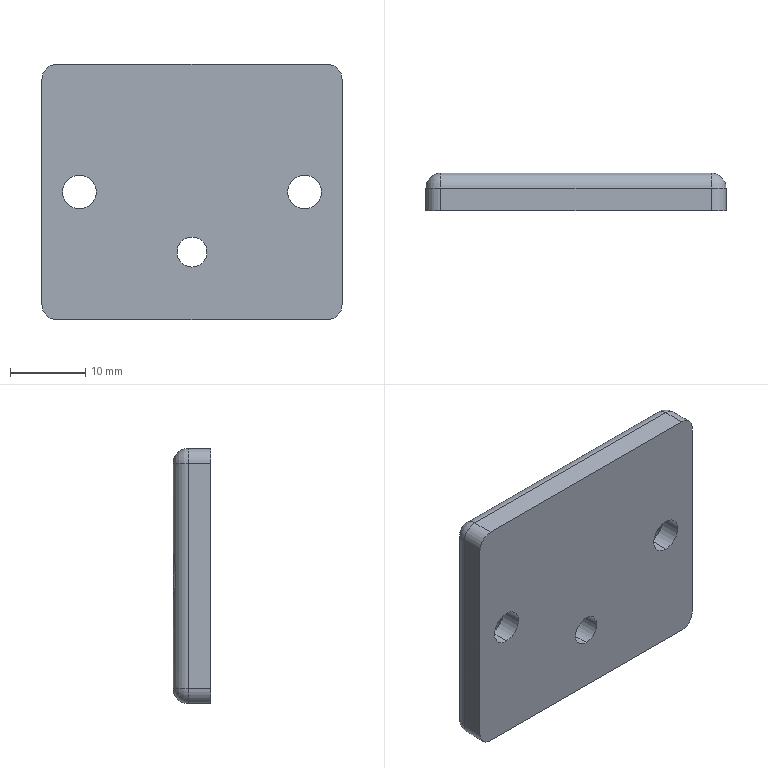Component | SolidWorks | 18ZTJ-NVT-01-006-1 | 1 solid | 28 faces | box 40 x 5 x 34 mm | volume 6347 mm3 | cylinder 14 | plane 6 | cone 4 | sphere 4 | commonest cylinder face diameters 4 x10 4.5 x4 | material #45
STEP:
#1=COLOUR_RGB('',0.7922,0.8196,0.9333);
#2=FILL_AREA_STYLE_COLOUR('',#1);
#3=FILL_AREA_STYLE('',(#2));
#4=SURFACE_STYLE_FILL_AREA(#3);
#5=SURFACE_SIDE_STYLE('',(#4));
#6=SURFACE_STYLE_USAGE(.BOTH.,#5);
#7=PRESENTATION_STYLE_ASSIGNMENT((#6));
#8=CARTESIAN_POINT('',(-0.5354,0.3728,3.583));
#9=VERTEX_POINT('',#8);
#10=CARTESIAN_POINT('',(-0.5354,0.3728,3.74));
#11=VERTEX_POINT('',#10);
#12=CARTESIAN_POINT('',(-0.5354,0.3728,3.661));
#13=DIRECTION('',(0.,1.,0.));
#14=DIRECTION('',(0.,0.,1.));
#15=AXIS2_PLACEMENT_3D('',#12,#13,#14);
#16=CIRCLE('',#15,0.07874);
#17=EDGE_CURVE('',#9,#11,#16,.T.);
#18=ORIENTED_EDGE('',*,*,#17,.F.);
#19=CARTESIAN_POINT('',(-0.5354,0.5697,3.583));
#20=VERTEX_POINT('',#19);
#21=CARTESIAN_POINT('',(-0.5354,0.5697,3.583));
#22=DIRECTION('',(0.,1.,0.));
#23=VECTOR('',#22,39.37);
#24=LINE('',#21,#23);
#25=EDGE_CURVE('',#9,#20,#24,.T.);
#26=ORIENTED_EDGE('',*,*,#25,.T.);
#27=CARTESIAN_POINT('',(-0.5354,0.5697,3.74));
#28=VERTEX_POINT('',#27);
#29=CARTESIAN_POINT('',(-0.5354,0.5697,3.661));
#30=DIRECTION('',(0.,1.,0.));
#31=DIRECTION('',(0.,0.,1.));
#32=AXIS2_PLACEMENT_3D('',#29,#30,#31);
#33=CIRCLE('',#32,0.07874);
#34=EDGE_CURVE('',#20,#28,#33,.T.);
#35=ORIENTED_EDGE('',*,*,#34,.T.);
#36=CARTESIAN_POINT('',(-0.5354,0.5697,3.74));
#37=DIRECTION('',(0.,1.,0.));
#38=VECTOR('',#37,39.37);
#39=LINE('',#36,#38);
#40=EDGE_CURVE('',#11,#28,#39,.T.);
#41=ORIENTED_EDGE('',*,*,#40,.F.);
#42=EDGE_LOOP('',(#18,#26,#35,#41));
#43=FACE_OUTER_BOUND('',#42,.T.);
#44=CARTESIAN_POINT('',(-0.5354,0.5697,3.661));
#45=DIRECTION('',(0.,1.,0.));
#46=DIRECTION('',(0.,0.,1.));
#47=AXIS2_PLACEMENT_3D('',#44,#45,#46);
#48=CYLINDRICAL_SURFACE('',#47,0.07874);
#49=ADVANCED_FACE('',(#43),#48,.F.);
#50=CARTESIAN_POINT('',(-1.126,0.4819,3.888));
#51=VERTEX_POINT('',#50);
#52=CARTESIAN_POINT('',(-1.126,0.4819,4.065));
#53=VERTEX_POINT('',#52);
#54=CARTESIAN_POINT('',(-1.126,0.4819,3.976));
#55=DIRECTION('',(0.,1.,0.));
#56=DIRECTION('',(0.,0.,1.));
#57=AXIS2_PLACEMENT_3D('',#54,#55,#56);
#58=CIRCLE('',#57,0.08858);
#59=EDGE_CURVE('',#51,#53,#58,.T.);
#60=ORIENTED_EDGE('',*,*,#59,.F.);
#61=CARTESIAN_POINT('',(-1.126,0.5697,3.8));
#62=VERTEX_POINT('',#61);
#63=CARTESIAN_POINT('',(-1.126,0.5697,3.8));
#64=DIRECTION('',(0.,0.7071,-0.7071));
#65=VECTOR('',#64,39.37);
#66=LINE('',#63,#65);
#67=EDGE_CURVE('',#51,#62,#66,.T.);
#68=ORIENTED_EDGE('',*,*,#67,.T.);
#69=CARTESIAN_POINT('',(-1.244,0.5697,3.845));
#70=VERTEX_POINT('',#69);
#71=CARTESIAN_POINT('',(-1.126,0.5697,3.976));
#72=DIRECTION('',(0.,1.,0.));
#73=DIRECTION('',(0.,0.,1.));
#74=AXIS2_PLACEMENT_3D('',#71,#72,#73);
#75=CIRCLE('',#74,0.1764);
#76=EDGE_CURVE('',#62,#70,#75,.T.);
#77=ORIENTED_EDGE('',*,*,#76,.T.);
#78=CARTESIAN_POINT('',(-1.244,0.5697,4.107));
#79=VERTEX_POINT('',#78);
#80=CARTESIAN_POINT('',(-1.244,0.5697,3.845));
#81=CARTESIAN_POINT('',(-1.249,0.5697,3.849));
#82=CARTESIAN_POINT('',(-1.253,0.5693,3.854));
#83=CARTESIAN_POINT('',(-1.26,0.5682,3.863));
#84=CARTESIAN_POINT('',(-1.263,0.5675,3.868));
#85=CARTESIAN_POINT('',(-1.268,0.5659,3.879));
#86=CARTESIAN_POINT('',(-1.271,0.565,3.884));
#87=CARTESIAN_POINT('',(-1.275,0.5633,3.895));
#88=CARTESIAN_POINT('',(-1.277,0.5624,3.901));
#89=CARTESIAN_POINT('',(-1.282,0.5599,3.917));
#90=CARTESIAN_POINT('',(-1.285,0.5585,3.929));
#91=CARTESIAN_POINT('',(-1.288,0.5565,3.953));
#92=CARTESIAN_POINT('',(-1.289,0.5559,3.964));
#93=CARTESIAN_POINT('',(-1.289,0.5559,3.988));
#94=CARTESIAN_POINT('',(-1.288,0.5565,4.));
#95=CARTESIAN_POINT('',(-1.285,0.5585,4.024));
#96=CARTESIAN_POINT('',(-1.282,0.5599,4.035));
#97=CARTESIAN_POINT('',(-1.277,0.5624,4.052));
#98=CARTESIAN_POINT('',(-1.275,0.5632,4.057));
#99=CARTESIAN_POINT('',(-1.271,0.565,4.068));
#100=CARTESIAN_POINT('',(-1.268,0.5659,4.074));
#101=CARTESIAN_POINT('',(-1.263,0.5675,4.084));
#102=CARTESIAN_POINT('',(-1.26,0.5682,4.089));
#103=CARTESIAN_POINT('',(-1.253,0.5693,4.099));
#104=CARTESIAN_POINT('',(-1.249,0.5697,4.103));
#105=CARTESIAN_POINT('',(-1.244,0.5697,4.107));
#106=B_SPLINE_CURVE_WITH_KNOTS('',3,(#80,#81,#82,#83,#84,#85,#86,#87,#88,#89,#90,#91,#92,#93,#94,#95,#96,#97,#98,#99,#100,#101,#102,#103,#104,#105),.UNSPECIFIED.,.F.,.F.,(4,2,2,2,2,2,2,2,2,2,2,2,4),(0.,0.000451,0.000902,0.001353,0.001804,0.002706,0.003608,0.00451,0.005412,0.005863,0.006314,0.006765,0.007216),.UNSPECIFIED.);
#107=EDGE_CURVE('',#70,#79,#106,.T.);
#108=ORIENTED_EDGE('',*,*,#107,.T.);
#109=CARTESIAN_POINT('',(-1.126,0.5697,4.153));
#110=VERTEX_POINT('',#109);
#111=CARTESIAN_POINT('',(-1.126,0.5697,3.976));
#112=DIRECTION('',(0.,1.,0.));
#113=DIRECTION('',(0.,0.,1.));
#114=AXIS2_PLACEMENT_3D('',#111,#112,#113);
#115=CIRCLE('',#114,0.1764);
#116=EDGE_CURVE('',#79,#110,#115,.T.);
#117=ORIENTED_EDGE('',*,*,#116,.T.);
#118=CARTESIAN_POINT('',(-1.126,0.5697,4.153));
#119=DIRECTION('',(0.,0.7071,0.7071));
#120=VECTOR('',#119,39.37);
#121=LINE('',#118,#120);
#122=EDGE_CURVE('',#53,#110,#121,.T.);
#123=ORIENTED_EDGE('',*,*,#122,.F.);
#124=EDGE_LOOP('',(#60,#68,#77,#108,#117,#123));
#125=FACE_OUTER_BOUND('',#124,.T.);
#126=CARTESIAN_POINT('',(-1.126,0.5697,3.976));
#127=DIRECTION('',(0.,1.,0.));
#128=DIRECTION('',(0.,0.,1.));
#129=AXIS2_PLACEMENT_3D('',#126,#127,#128);
#130=CONICAL_SURFACE('',#129,0.1764,0.7854);
#131=ADVANCED_FACE('',(#125),#130,.F.);
#132=CARTESIAN_POINT('',(-1.126,0.3728,3.888));
#133=VERTEX_POINT('',#132);
#134=CARTESIAN_POINT('',(-1.126,0.3728,4.065));
#135=VERTEX_POINT('',#134);
#136=CARTESIAN_POINT('',(-1.126,0.3728,3.976));
#137=DIRECTION('',(0.,1.,0.));
#138=DIRECTION('',(0.,0.,1.));
#139=AXIS2_PLACEMENT_3D('',#136,#137,#138);
#140=CIRCLE('',#139,0.08858);
#141=EDGE_CURVE('',#133,#135,#140,.T.);
#142=ORIENTED_EDGE('',*,*,#141,.F.);
#143=CARTESIAN_POINT('',(-1.126,0.5697,3.888));
#144=DIRECTION('',(0.,1.,0.));
#145=VECTOR('',#144,39.37);
#146=LINE('',#143,#145);
#147=EDGE_CURVE('',#133,#51,#146,.T.);
#148=ORIENTED_EDGE('',*,*,#147,.T.);
#149=ORIENTED_EDGE('',*,*,#59,.T.);
#150=CARTESIAN_POINT('',(-1.126,0.5697,4.065));
#151=DIRECTION('',(0.,1.,0.));
#152=VECTOR('',#151,39.37);
#153=LINE('',#150,#152);
#154=EDGE_CURVE('',#135,#53,#153,.T.);
#155=ORIENTED_EDGE('',*,*,#154,.F.);
#156=EDGE_LOOP('',(#142,#148,#149,#155));
#157=FACE_OUTER_BOUND('',#156,.T.);
#158=CARTESIAN_POINT('',(-1.126,0.5697,3.976));
#159=DIRECTION('',(0.,1.,0.));
#160=DIRECTION('',(0.,0.,1.));
#161=AXIS2_PLACEMENT_3D('',#158,#159,#160);
#162=CYLINDRICAL_SURFACE('',#161,0.08858);
#163=ADVANCED_FACE('',(#157),#162,.F.);
#164=CARTESIAN_POINT('',(0.05513,0.4819,3.888));
#165=VERTEX_POINT('',#164);
#166=CARTESIAN_POINT('',(0.05513,0.4819,4.065));
#167=VERTEX_POINT('',#166);
#168=CARTESIAN_POINT('',(0.05513,0.4819,3.976));
#169=DIRECTION('',(0.,1.,0.));
#170=DIRECTION('',(0.,0.,1.));
#171=AXIS2_PLACEMENT_3D('',#168,#169,#170);
#172=CIRCLE('',#171,0.08858);
#173=EDGE_CURVE('',#165,#167,#172,.T.);
#174=ORIENTED_EDGE('',*,*,#173,.F.);
#175=CARTESIAN_POINT('',(0.05513,0.5697,3.8));
#176=VERTEX_POINT('',#175);
#177=CARTESIAN_POINT('',(0.05513,0.5697,3.8));
#178=DIRECTION('',(0.,0.7071,-0.7071));
#179=VECTOR('',#178,39.37);
#180=LINE('',#177,#179);
#181=EDGE_CURVE('',#165,#176,#180,.T.);
#182=ORIENTED_EDGE('',*,*,#181,.T.);
#183=CARTESIAN_POINT('',(0.05513,0.5697,4.153));
#184=VERTEX_POINT('',#183);
#185=CARTESIAN_POINT('',(0.05513,0.5697,3.976));
#186=DIRECTION('',(0.,1.,0.));
#187=DIRECTION('',(0.,0.,1.));
#188=AXIS2_PLACEMENT_3D('',#185,#186,#187);
#189=CIRCLE('',#188,0.1764);
#190=EDGE_CURVE('',#176,#184,#189,.T.);
#191=ORIENTED_EDGE('',*,*,#190,.T.);
#192=CARTESIAN_POINT('',(0.05513,0.5697,4.153));
#193=DIRECTION('',(0.,0.7071,0.7071));
#194=VECTOR('',#193,39.37);
#195=LINE('',#192,#194);
#196=EDGE_CURVE('',#167,#184,#195,.T.);
#197=ORIENTED_EDGE('',*,*,#196,.F.);
#198=EDGE_LOOP('',(#174,#182,#191,#197));
#199=FACE_OUTER_BOUND('',#198,.T.);
#200=CARTESIAN_POINT('',(0.05513,0.5697,3.976));
#201=DIRECTION('',(0.,1.,0.));
#202=DIRECTION('',(0.,0.,1.));
#203=AXIS2_PLACEMENT_3D('',#200,#201,#202);
#204=CONICAL_SURFACE('',#203,0.1764,0.7854);
#205=ADVANCED_FACE('',(#199),#204,.F.);
#206=CARTESIAN_POINT('',(0.05513,0.3728,3.888));
#207=VERTEX_POINT('',#206);
#208=CARTESIAN_POINT('',(0.05513,0.3728,4.065));
#209=VERTEX_POINT('',#208);
#210=CARTESIAN_POINT('',(0.05513,0.3728,3.976));
#211=DIRECTION('',(0.,1.,0.));
#212=DIRECTION('',(0.,0.,1.));
#213=AXIS2_PLACEMENT_3D('',#210,#211,#212);
#214=CIRCLE('',#213,0.08858);
#215=EDGE_CURVE('',#207,#209,#214,.T.);
#216=ORIENTED_EDGE('',*,*,#215,.F.);
#217=CARTESIAN_POINT('',(0.05513,0.5697,3.888));
#218=DIRECTION('',(0.,1.,0.));
#219=VECTOR('',#218,39.37);
#220=LINE('',#217,#219);
#221=EDGE_CURVE('',#207,#165,#220,.T.);
#222=ORIENTED_EDGE('',*,*,#221,.T.);
#223=ORIENTED_EDGE('',*,*,#173,.T.);
#224=CARTESIAN_POINT('',(0.05513,0.5697,4.065));
#225=DIRECTION('',(0.,1.,0.));
#226=VECTOR('',#225,39.37);
#227=LINE('',#224,#226);
#228=EDGE_CURVE('',#209,#167,#227,.T.);
#229=ORIENTED_EDGE('',*,*,#228,.F.);
#230=EDGE_LOOP('',(#216,#222,#223,#229));
#231=FACE_OUTER_BOUND('',#230,.T.);
#232=CARTESIAN_POINT('',(0.05513,0.5697,3.976));
#233=DIRECTION('',(0.,1.,0.));
#234=DIRECTION('',(0.,0.,1.));
#235=AXIS2_PLACEMENT_3D('',#232,#233,#234);
#236=CYLINDRICAL_SURFACE('',#235,0.08858);
#237=ADVANCED_FACE('',(#231),#236,.F.);
#238=CARTESIAN_POINT('',(-1.323,0.491,4.567));
#239=VERTEX_POINT('',#238);
#240=CARTESIAN_POINT('',(-1.323,0.491,3.386));
#241=VERTEX_POINT('',#240);
#242=CARTESIAN_POINT('',(-1.323,0.491,4.646));
#243=DIRECTION('',(0.,0.,-1.));
#244=VECTOR('',#243,39.37);
#245=LINE('',#242,#244);
#246=EDGE_CURVE('',#239,#241,#245,.T.);
#247=ORIENTED_EDGE('',*,*,#246,.T.);
#248=CARTESIAN_POINT('',(-1.323,0.3728,3.386));
#249=VERTEX_POINT('',#248);
#250=CARTESIAN_POINT('',(-1.323,0.5697,3.386));
#251=DIRECTION('',(0.,-1.,0.));
#252=VECTOR('',#251,39.37);
#253=LINE('',#250,#252);
#254=EDGE_CURVE('',#241,#249,#253,.T.);
#255=ORIENTED_EDGE('',*,*,#254,.T.);
#256=CARTESIAN_POINT('',(-1.323,0.3728,4.567));
#257=VERTEX_POINT('',#256);
#258=CARTESIAN_POINT('',(-1.323,0.3728,4.646));
#259=DIRECTION('',(0.,0.,1.));
#260=VECTOR('',#259,39.37);
#261=LINE('',#258,#260);
#262=EDGE_CURVE('',#249,#257,#261,.T.);
#263=ORIENTED_EDGE('',*,*,#262,.T.);
#264=CARTESIAN_POINT('',(-1.323,0.5697,4.567));
#265=DIRECTION('',(0.,1.,0.));
#266=VECTOR('',#265,39.37);
#267=LINE('',#264,#266);
#268=EDGE_CURVE('',#257,#239,#267,.T.);
#269=ORIENTED_EDGE('',*,*,#268,.T.);
#270=EDGE_LOOP('',(#247,#255,#263,#269));
#271=FACE_OUTER_BOUND('',#270,.T.);
#272=CARTESIAN_POINT('',(-1.323,0.5697,4.646));
#273=DIRECTION('',(1.,0.,0.));
#274=DIRECTION('',(0.,0.,-1.));
#275=AXIS2_PLACEMENT_3D('',#272,#273,#274);
#276=PLANE('',#275);
#277=ADVANCED_FACE('',(#271),#276,.F.);
#278=CARTESIAN_POINT('',(0.1732,0.491,4.646));
#279=VERTEX_POINT('',#278);
#280=CARTESIAN_POINT('',(-1.244,0.491,4.646));
#281=VERTEX_POINT('',#280);
#282=CARTESIAN_POINT('',(-1.323,0.491,4.646));
#283=DIRECTION('',(-1.,0.,0.));
#284=VECTOR('',#283,39.37);
#285=LINE('',#282,#284);
#286=EDGE_CURVE('',#279,#281,#285,.T.);
#287=ORIENTED_EDGE('',*,*,#286,.T.);
#288=CARTESIAN_POINT('',(-1.244,0.3728,4.646));
#289=VERTEX_POINT('',#288);
#290=CARTESIAN_POINT('',(-1.244,0.5697,4.646));
#291=DIRECTION('',(0.,-1.,0.));
#292=VECTOR('',#291,39.37);
#293=LINE('',#290,#292);
#294=EDGE_CURVE('',#281,#289,#293,.T.);
#295=ORIENTED_EDGE('',*,*,#294,.T.);
#296=CARTESIAN_POINT('',(0.1732,0.3728,4.646));
#297=VERTEX_POINT('',#296);
#298=CARTESIAN_POINT('',(-1.323,0.3728,4.646));
#299=DIRECTION('',(1.,0.,0.));
#300=VECTOR('',#299,39.37);
#301=LINE('',#298,#300);
#302=EDGE_CURVE('',#289,#297,#301,.T.);
#303=ORIENTED_EDGE('',*,*,#302,.T.);
#304=CARTESIAN_POINT('',(0.1732,0.5697,4.646));
#305=DIRECTION('',(0.,1.,0.));
#306=VECTOR('',#305,39.37);
#307=LINE('',#304,#306);
#308=EDGE_CURVE('',#297,#279,#307,.T.);
#309=ORIENTED_EDGE('',*,*,#308,.T.);
#310=EDGE_LOOP('',(#287,#295,#303,#309));
#311=FACE_OUTER_BOUND('',#310,.T.);
#312=CARTESIAN_POINT('',(-1.323,0.5697,4.646));
#313=DIRECTION('',(0.,0.,-1.));
#314=DIRECTION('',(-1.,0.,0.));
#315=AXIS2_PLACEMENT_3D('',#312,#313,#314);
#316=PLANE('',#315);
#317=ADVANCED_FACE('',(#311),#316,.F.);
#318=CARTESIAN_POINT('',(0.252,0.3728,4.567));
#319=VERTEX_POINT('',#318);
#320=CARTESIAN_POINT('',(0.252,0.3728,3.386));
#321=VERTEX_POINT('',#320);
#322=CARTESIAN_POINT('',(0.252,0.3728,4.646));
#323=DIRECTION('',(0.,0.,-1.));
#324=VECTOR('',#323,39.37);
#325=LINE('',#322,#324);
#326=EDGE_CURVE('',#319,#321,#325,.T.);
#327=ORIENTED_EDGE('',*,*,#326,.T.);
#328=CARTESIAN_POINT('',(0.252,0.491,3.386));
#329=VERTEX_POINT('',#328);
#330=CARTESIAN_POINT('',(0.252,0.5697,3.386));
#331=DIRECTION('',(0.,1.,0.));
#332=VECTOR('',#331,39.37);
#333=LINE('',#330,#332);
#334=EDGE_CURVE('',#321,#329,#333,.T.);
#335=ORIENTED_EDGE('',*,*,#334,.T.);
#336=CARTESIAN_POINT('',(0.252,0.491,4.567));
#337=VERTEX_POINT('',#336);
#338=CARTESIAN_POINT('',(0.252,0.491,4.646));
#339=DIRECTION('',(0.,0.,1.));
#340=VECTOR('',#339,39.37);
#341=LINE('',#338,#340);
#342=EDGE_CURVE('',#329,#337,#341,.T.);
#343=ORIENTED_EDGE('',*,*,#342,.T.);
#344=CARTESIAN_POINT('',(0.252,0.5697,4.567));
#345=DIRECTION('',(0.,-1.,0.));
#346=VECTOR('',#345,39.37);
#347=LINE('',#344,#346);
#348=EDGE_CURVE('',#337,#319,#347,.T.);
#349=ORIENTED_EDGE('',*,*,#348,.T.);
#350=EDGE_LOOP('',(#327,#335,#343,#349));
#351=FACE_OUTER_BOUND('',#350,.T.);
#352=CARTESIAN_POINT('',(0.252,0.5697,4.646));
#353=DIRECTION('',(-1.,0.,0.));
#354=DIRECTION('',(0.,0.,1.));
#355=AXIS2_PLACEMENT_3D('',#352,#353,#354);
#356=PLANE('',#355);
#357=ADVANCED_FACE('',(#351),#356,.F.);
#358=CARTESIAN_POINT('',(0.1732,0.3728,3.307));
#359=VERTEX_POINT('',#358);
#360=CARTESIAN_POINT('',(-1.244,0.3728,3.307));
#361=VERTEX_POINT('',#360);
#362=CARTESIAN_POINT('',(-1.323,0.3728,3.307));
#363=DIRECTION('',(-1.,0.,0.));
#364=VECTOR('',#363,39.37);
#365=LINE('',#362,#364);
#366=EDGE_CURVE('',#359,#361,#365,.T.);
#367=ORIENTED_EDGE('',*,*,#366,.T.);
#368=CARTESIAN_POINT('',(-1.244,0.491,3.307));
#369=VERTEX_POINT('',#368);
#370=CARTESIAN_POINT('',(-1.244,0.5697,3.307));
#371=DIRECTION('',(0.,1.,0.));
#372=VECTOR('',#371,39.37);
#373=LINE('',#370,#372);
#374=EDGE_CURVE('',#361,#369,#373,.T.);
#375=ORIENTED_EDGE('',*,*,#374,.T.);
#376=CARTESIAN_POINT('',(0.1732,0.491,3.307));
#377=VERTEX_POINT('',#376);
#378=CARTESIAN_POINT('',(-1.323,0.491,3.307));
#379=DIRECTION('',(1.,0.,0.));
#380=VECTOR('',#379,39.37);
#381=LINE('',#378,#380);
#382=EDGE_CURVE('',#369,#377,#381,.T.);
#383=ORIENTED_EDGE('',*,*,#382,.T.);
#384=CARTESIAN_POINT('',(0.1732,0.5697,3.307));
#385=DIRECTION('',(0.,-1.,0.));
#386=VECTOR('',#385,39.37);
#387=LINE('',#384,#386);
#388=EDGE_CURVE('',#377,#359,#387,.T.);
#389=ORIENTED_EDGE('',*,*,#388,.T.);
#390=EDGE_LOOP('',(#367,#375,#383,#389));
#391=FACE_OUTER_BOUND('',#390,.T.);
#392=CARTESIAN_POINT('',(-1.323,0.5697,3.307));
#393=DIRECTION('',(0.,0.,1.));
#394=DIRECTION('',(1.,0.,0.));
#395=AXIS2_PLACEMENT_3D('',#392,#393,#394);
#396=PLANE('',#395);
#397=ADVANCED_FACE('',(#391),#396,.F.);
#398=CARTESIAN_POINT('',(-0.5354,0.5697,3.661));
#399=DIRECTION('',(0.,1.,0.));
#400=DIRECTION('',(0.,0.,1.));
#401=AXIS2_PLACEMENT_3D('',#398,#399,#400);
#402=CIRCLE('',#401,0.07874);
#403=EDGE_CURVE('',#28,#20,#402,.T.);
#404=ORIENTED_EDGE('',*,*,#403,.F.);
#405=ORIENTED_EDGE('',*,*,#34,.F.);
#406=EDGE_LOOP('',(#404,#405));
#407=FACE_BOUND('',#406,.T.);
#408=ORIENTED_EDGE('',*,*,#116,.F.);
#409=CARTESIAN_POINT('',(-1.244,0.5697,4.567));
#410=VERTEX_POINT('',#409);
#411=CARTESIAN_POINT('',(-1.244,0.5697,4.646));
#412=DIRECTION('',(0.,0.,1.));
#413=VECTOR('',#412,39.37);
#414=LINE('',#411,#413);
#415=EDGE_CURVE('',#79,#410,#414,.T.);
#416=ORIENTED_EDGE('',*,*,#415,.T.);
#417=CARTESIAN_POINT('',(0.1732,0.5697,4.567));
#418=VERTEX_POINT('',#417);
#419=CARTESIAN_POINT('',(-1.323,0.5697,4.567));
#420=DIRECTION('',(1.,0.,0.));
#421=VECTOR('',#420,39.37);
#422=LINE('',#419,#421);
#423=EDGE_CURVE('',#410,#418,#422,.T.);
#424=ORIENTED_EDGE('',*,*,#423,.T.);
#425=CARTESIAN_POINT('',(0.1732,0.5697,4.107));
#426=VERTEX_POINT('',#425);
#427=CARTESIAN_POINT('',(0.1732,0.5697,4.646));
#428=DIRECTION('',(0.,0.,-1.));
#429=VECTOR('',#428,39.37);
#430=LINE('',#427,#429);
#431=EDGE_CURVE('',#418,#426,#430,.T.);
#432=ORIENTED_EDGE('',*,*,#431,.T.);
#433=CARTESIAN_POINT('',(0.05513,0.5697,3.976));
#434=DIRECTION('',(0.,1.,0.));
#435=DIRECTION('',(0.,0.,1.));
#436=AXIS2_PLACEMENT_3D('',#433,#434,#435);
#437=CIRCLE('',#436,0.1764);
#438=EDGE_CURVE('',#184,#426,#437,.T.);
#439=ORIENTED_EDGE('',*,*,#438,.F.);
#440=ORIENTED_EDGE('',*,*,#190,.F.);
#441=CARTESIAN_POINT('',(0.1732,0.5697,3.845));
#442=VERTEX_POINT('',#441);
#443=CARTESIAN_POINT('',(0.05513,0.5697,3.976));
#444=DIRECTION('',(0.,1.,0.));
#445=DIRECTION('',(0.,0.,1.));
#446=AXIS2_PLACEMENT_3D('',#443,#444,#445);
#447=CIRCLE('',#446,0.1764);
#448=EDGE_CURVE('',#442,#176,#447,.T.);
#449=ORIENTED_EDGE('',*,*,#448,.F.);
#450=CARTESIAN_POINT('',(0.1732,0.5697,3.386));
#451=VERTEX_POINT('',#450);
#452=CARTESIAN_POINT('',(0.1732,0.5697,4.646));
#453=DIRECTION('',(0.,0.,-1.));
#454=VECTOR('',#453,39.37);
#455=LINE('',#452,#454);
#456=EDGE_CURVE('',#442,#451,#455,.T.);
#457=ORIENTED_EDGE('',*,*,#456,.T.);
#458=CARTESIAN_POINT('',(-1.244,0.5697,3.386));
#459=VERTEX_POINT('',#458);
#460=CARTESIAN_POINT('',(-1.323,0.5697,3.386));
#461=DIRECTION('',(-1.,0.,0.));
#462=VECTOR('',#461,39.37);
#463=LINE('',#460,#462);
#464=EDGE_CURVE('',#451,#459,#463,.T.);
#465=ORIENTED_EDGE('',*,*,#464,.T.);
#466=CARTESIAN_POINT('',(-1.244,0.5697,4.646));
#467=DIRECTION('',(0.,0.,1.));
#468=VECTOR('',#467,39.37);
#469=LINE('',#466,#468);
#470=EDGE_CURVE('',#459,#70,#469,.T.);
#471=ORIENTED_EDGE('',*,*,#470,.T.);
#472=ORIENTED_EDGE('',*,*,#76,.F.);
#473=CARTESIAN_POINT('',(-1.126,0.5697,3.976));
#474=DIRECTION('',(0.,1.,0.));
#475=DIRECTION('',(0.,0.,1.));
#476=AXIS2_PLACEMENT_3D('',#473,#474,#475);
#477=CIRCLE('',#476,0.1764);
#478=EDGE_CURVE('',#110,#62,#477,.T.);
#479=ORIENTED_EDGE('',*,*,#478,.F.);
#480=EDGE_LOOP('',(#408,#416,#424,#432,#439,#440,#449,#457,#465,#471,#472,#479));
#481=FACE_OUTER_BOUND('',#480,.T.);
#482=CARTESIAN_POINT('',(-1.323,0.5697,4.646));
#483=DIRECTION('',(0.,-1.,0.));
#484=DIRECTION('',(0.,0.,-1.));
#485=AXIS2_PLACEMENT_3D('',#482,#483,#484);
#486=PLANE('',#485);
#487=ADVANCED_FACE('',(#407,#481),#486,.F.);
#488=CARTESIAN_POINT('',(-0.5354,0.3728,3.661));
#489=DIRECTION('',(0.,1.,0.));
#490=DIRECTION('',(0.,0.,1.));
#491=AXIS2_PLACEMENT_3D('',#488,#489,#490);
#492=CIRCLE('',#491,0.07874);
#493=EDGE_CURVE('',#11,#9,#492,.T.);
#494=ORIENTED_EDGE('',*,*,#493,.T.);
#495=ORIENTED_EDGE('',*,*,#17,.T.);
#496=EDGE_LOOP('',(#494,#495));
#497=FACE_BOUND('',#496,.T.);
#498=CARTESIAN_POINT('',(-1.126,0.3728,3.976));
#499=DIRECTION('',(0.,1.,0.));
#500=DIRECTION('',(0.,0.,1.));
#501=AXIS2_PLACEMENT_3D('',#498,#499,#500);
#502=CIRCLE('',#501,0.08858);
#503=EDGE_CURVE('',#135,#133,#502,.T.);
#504=ORIENTED_EDGE('',*,*,#503,.T.);
#505=ORIENTED_EDGE('',*,*,#141,.T.);
#506=EDGE_LOOP('',(#504,#505));
#507=FACE_BOUND('',#506,.T.);
#508=CARTESIAN_POINT('',(0.05513,0.3728,3.976));
#509=DIRECTION('',(0.,1.,0.));
#510=DIRECTION('',(0.,0.,1.));
#511=AXIS2_PLACEMENT_3D('',#508,#509,#510);
#512=CIRCLE('',#511,0.08858);
#513=EDGE_CURVE('',#209,#207,#512,.T.);
#514=ORIENTED_EDGE('',*,*,#513,.T.);
#515=ORIENTED_EDGE('',*,*,#215,.T.);
#516=EDGE_LOOP('',(#514,#515));
#517=FACE_BOUND('',#516,.T.);
#518=ORIENTED_EDGE('',*,*,#262,.F.);
#519=CARTESIAN_POINT('',(-1.244,0.3728,3.386));
#520=DIRECTION('',(0.,-1.,0.));
#521=DIRECTION('',(0.,0.,-1.));
#522=AXIS2_PLACEMENT_3D('',#519,#520,#521);
#523=CIRCLE('',#522,0.07874);
#524=EDGE_CURVE('',#249,#361,#523,.T.);
#525=ORIENTED_EDGE('',*,*,#524,.T.);
#526=ORIENTED_EDGE('',*,*,#366,.F.);
#527=CARTESIAN_POINT('',(0.1732,0.3728,3.386));
#528=DIRECTION('',(0.,-1.,0.));
#529=DIRECTION('',(0.,0.,-1.));
#530=AXIS2_PLACEMENT_3D('',#527,#528,#529);
#531=CIRCLE('',#530,0.07874);
#532=EDGE_CURVE('',#359,#321,#531,.T.);
#533=ORIENTED_EDGE('',*,*,#532,.T.);
#534=ORIENTED_EDGE('',*,*,#326,.F.);
#535=CARTESIAN_POINT('',(0.1732,0.3728,4.567));
#536=DIRECTION('',(0.,-1.,0.));
#537=DIRECTION('',(0.,0.,-1.));
#538=AXIS2_PLACEMENT_3D('',#535,#536,#537);
#539=CIRCLE('',#538,0.07874);
#540=EDGE_CURVE('',#319,#297,#539,.T.);
#541=ORIENTED_EDGE('',*,*,#540,.T.);
#542=ORIENTED_EDGE('',*,*,#302,.F.);
#543=CARTESIAN_POINT('',(-1.244,0.3728,4.567));
#544=DIRECTION('',(0.,-1.,0.));
#545=DIRECTION('',(0.,0.,-1.));
#546=AXIS2_PLACEMENT_3D('',#543,#544,#545);
#547=CIRCLE('',#546,0.07874);
#548=EDGE_CURVE('',#289,#257,#547,.T.);
#549=ORIENTED_EDGE('',*,*,#548,.T.);
#550=EDGE_LOOP('',(#518,#525,#526,#533,#534,#541,#542,#549));
#551=FACE_OUTER_BOUND('',#550,.T.);
#552=CARTESIAN_POINT('',(-1.323,0.3728,4.646));
#553=DIRECTION('',(0.,-1.,0.));
#554=DIRECTION('',(0.,0.,-1.));
#555=AXIS2_PLACEMENT_3D('',#552,#553,#554);
#556=PLANE('',#555);
#557=ADVANCED_FACE('',(#497,#507,#517,#551),#556,.T.);
#558=ORIENTED_EDGE('',*,*,#221,.F.);
#559=ORIENTED_EDGE('',*,*,#513,.F.);
#560=ORIENTED_EDGE('',*,*,#228,.T.);
#561=CARTESIAN_POINT('',(0.05513,0.4819,3.976));
#562=DIRECTION('',(0.,1.,0.));
#563=DIRECTION('',(0.,0.,1.));
#564=AXIS2_PLACEMENT_3D('',#561,#562,#563);
#565=CIRCLE('',#564,0.08858);
#566=EDGE_CURVE('',#167,#165,#565,.T.);
#567=ORIENTED_EDGE('',*,*,#566,.T.);
#568=EDGE_LOOP('',(#558,#559,#560,#567));
#569=FACE_OUTER_BOUND('',#568,.T.);
#570=CARTESIAN_POINT('',(0.05513,0.5697,3.976));
#571=DIRECTION('',(0.,1.,0.));
#572=DIRECTION('',(0.,0.,1.));
#573=AXIS2_PLACEMENT_3D('',#570,#571,#572);
#574=CYLINDRICAL_SURFACE('',#573,0.08858);
#575=ADVANCED_FACE('',(#569),#574,.F.);
#576=ORIENTED_EDGE('',*,*,#181,.F.);
#577=ORIENTED_EDGE('',*,*,#566,.F.);
#578=ORIENTED_EDGE('',*,*,#196,.T.);
#579=ORIENTED_EDGE('',*,*,#438,.T.);
#580=CARTESIAN_POINT('',(0.1732,0.5697,4.107));
#581=CARTESIAN_POINT('',(0.1778,0.5697,4.103));
#582=CARTESIAN_POINT('',(0.1817,0.5693,4.099));
#583=CARTESIAN_POINT('',(0.1887,0.5682,4.089));
#584=CARTESIAN_POINT('',(0.1919,0.5675,4.084));
#585=CARTESIAN_POINT('',(0.1976,0.5659,4.074));
#586=CARTESIAN_POINT('',(0.2001,0.565,4.069));
#587=CARTESIAN_POINT('',(0.2045,0.5633,4.058));
#588=CARTESIAN_POINT('',(0.2064,0.5624,4.052));
#589=CARTESIAN_POINT('',(0.2114,0.5599,4.035));
#590=CARTESIAN_POINT('',(0.2138,0.5585,4.024));
#591=CARTESIAN_POINT('',(0.217,0.5565,4.));
#592=CARTESIAN_POINT('',(0.2177,0.5559,3.988));
#593=CARTESIAN_POINT('',(0.2177,0.5559,3.965));
#594=CARTESIAN_POINT('',(0.217,0.5565,3.953));
#595=CARTESIAN_POINT('',(0.2138,0.5585,3.929));
#596=CARTESIAN_POINT('',(0.2114,0.5599,3.918));
#597=CARTESIAN_POINT('',(0.2065,0.5624,3.901));
#598=CARTESIAN_POINT('',(0.2046,0.5632,3.895));
#599=CARTESIAN_POINT('',(0.2002,0.565,3.884));
#600=CARTESIAN_POINT('',(0.1977,0.5659,3.879));
#601=CARTESIAN_POINT('',(0.192,0.5675,3.869));
#602=CARTESIAN_POINT('',(0.1889,0.5682,3.863));
#603=CARTESIAN_POINT('',(0.1817,0.5693,3.854));
#604=CARTESIAN_POINT('',(0.1777,0.5697,3.849));
#605=CARTESIAN_POINT('',(0.1732,0.5697,3.845));
#606=B_SPLINE_CURVE_WITH_KNOTS('',3,(#580,#581,#582,#583,#584,#585,#586,#587,#588,#589,#590,#591,#592,#593,#594,#595,#596,#597,#598,#599,#600,#601,#602,#603,#604,#605),.UNSPECIFIED.,.F.,.F.,(4,2,2,2,2,2,2,2,2,2,2,2,4),(0.,0.000451,0.000902,0.001353,0.001804,0.002706,0.003608,0.00451,0.005412,0.005863,0.006314,0.006765,0.007216),.UNSPECIFIED.);
#607=EDGE_CURVE('',#426,#442,#606,.T.);
#608=ORIENTED_EDGE('',*,*,#607,.T.);
#609=ORIENTED_EDGE('',*,*,#448,.T.);
#610=EDGE_LOOP('',(#576,#577,#578,#579,#608,#609));
#611=FACE_OUTER_BOUND('',#610,.T.);
#612=CARTESIAN_POINT('',(0.05513,0.5697,3.976));
#613=DIRECTION('',(0.,1.,0.));
#614=DIRECTION('',(0.,0.,1.));
#615=AXIS2_PLACEMENT_3D('',#612,#613,#614);
#616=CONICAL_SURFACE('',#615,0.1764,0.7854);
#617=ADVANCED_FACE('',(#611),#616,.F.);
#618=ORIENTED_EDGE('',*,*,#147,.F.);
#619=ORIENTED_EDGE('',*,*,#503,.F.);
#620=ORIENTED_EDGE('',*,*,#154,.T.);
#621=CARTESIAN_POINT('',(-1.126,0.4819,3.976));
#622=DIRECTION('',(0.,1.,0.));
#623=DIRECTION('',(0.,0.,1.));
#624=AXIS2_PLACEMENT_3D('',#621,#622,#623);
#625=CIRCLE('',#624,0.08858);
#626=EDGE_CURVE('',#53,#51,#625,.T.);
#627=ORIENTED_EDGE('',*,*,#626,.T.);
#628=EDGE_LOOP('',(#618,#619,#620,#627));
#629=FACE_OUTER_BOUND('',#628,.T.);
#630=CARTESIAN_POINT('',(-1.126,0.5697,3.976));
#631=DIRECTION('',(0.,1.,0.));
#632=DIRECTION('',(0.,0.,1.));
#633=AXIS2_PLACEMENT_3D('',#630,#631,#632);
#634=CYLINDRICAL_SURFACE('',#633,0.08858);
#635=ADVANCED_FACE('',(#629),#634,.F.);
#636=ORIENTED_EDGE('',*,*,#67,.F.);
#637=ORIENTED_EDGE('',*,*,#626,.F.);
#638=ORIENTED_EDGE('',*,*,#122,.T.);
#639=ORIENTED_EDGE('',*,*,#478,.T.);
#640=EDGE_LOOP('',(#636,#637,#638,#639));
#641=FACE_OUTER_BOUND('',#640,.T.);
#642=CARTESIAN_POINT('',(-1.126,0.5697,3.976));
#643=DIRECTION('',(0.,1.,0.));
#644=DIRECTION('',(0.,0.,1.));
#645=AXIS2_PLACEMENT_3D('',#642,#643,#644);
#646=CONICAL_SURFACE('',#645,0.1764,0.7854);
#647=ADVANCED_FACE('',(#641),#646,.F.);
#648=ORIENTED_EDGE('',*,*,#524,.F.);
#649=ORIENTED_EDGE('',*,*,#254,.F.);
#650=CARTESIAN_POINT('',(-1.244,0.491,3.386));
#651=DIRECTION('',(0.,1.,0.));
#652=DIRECTION('',(0.,0.,1.));
#653=AXIS2_PLACEMENT_3D('',#650,#651,#652);
#654=CIRCLE('',#653,0.07874);
#655=EDGE_CURVE('',#369,#241,#654,.T.);
#656=ORIENTED_EDGE('',*,*,#655,.F.);
#657=ORIENTED_EDGE('',*,*,#374,.F.);
#658=EDGE_LOOP('',(#648,#649,#656,#657));
#659=FACE_OUTER_BOUND('',#658,.T.);
#660=CARTESIAN_POINT('',(-1.244,0.5697,3.386));
#661=DIRECTION('',(0.,-1.,0.));
#662=DIRECTION('',(0.,0.,-1.));
#663=AXIS2_PLACEMENT_3D('',#660,#661,#662);
#664=CYLINDRICAL_SURFACE('',#663,0.07874);
#665=ADVANCED_FACE('',(#659),#664,.T.);
#666=CARTESIAN_POINT('',(0.1732,0.491,3.386));
#667=DIRECTION('',(1.,0.,0.));
#668=DIRECTION('',(0.,0.,-1.));
#669=AXIS2_PLACEMENT_3D('',#666,#667,#668);
#670=CIRCLE('',#669,0.07874);
#671=EDGE_CURVE('',#377,#451,#670,.T.);
#672=ORIENTED_EDGE('',*,*,#671,.F.);
#673=ORIENTED_EDGE('',*,*,#382,.F.);
#674=CARTESIAN_POINT('',(-1.244,0.491,3.386));
#675=DIRECTION('',(-1.,0.,0.));
#676=DIRECTION('',(0.,0.,1.));
#677=AXIS2_PLACEMENT_3D('',#674,#675,#676);
#678=CIRCLE('',#677,0.07874);
#679=EDGE_CURVE('',#459,#369,#678,.T.);
#680=ORIENTED_EDGE('',*,*,#679,.F.);
#681=ORIENTED_EDGE('',*,*,#464,.F.);
#682=EDGE_LOOP('',(#672,#673,#680,#681));
#683=FACE_OUTER_BOUND('',#682,.T.);
#684=CARTESIAN_POINT('',(-1.323,0.491,3.386));
#685=DIRECTION('',(-1.,0.,0.));
#686=DIRECTION('',(0.,0.,1.));
#687=AXIS2_PLACEMENT_3D('',#684,#685,#686);
#688=CYLINDRICAL_SURFACE('',#687,0.07874);
#689=ADVANCED_FACE('',(#683),#688,.T.);
#690=ORIENTED_EDGE('',*,*,#532,.F.);
#691=ORIENTED_EDGE('',*,*,#388,.F.);
#692=CARTESIAN_POINT('',(0.1732,0.491,3.386));
#693=DIRECTION('',(0.,1.,0.));
#694=DIRECTION('',(0.,0.,1.));
#695=AXIS2_PLACEMENT_3D('',#692,#693,#694);
#696=CIRCLE('',#695,0.07874);
#697=EDGE_CURVE('',#329,#377,#696,.T.);
#698=ORIENTED_EDGE('',*,*,#697,.F.);
#699=ORIENTED_EDGE('',*,*,#334,.F.);
#700=EDGE_LOOP('',(#690,#691,#698,#699));
#701=FACE_OUTER_BOUND('',#700,.T.);
#702=CARTESIAN_POINT('',(0.1732,0.5697,3.386));
#703=DIRECTION('',(0.,-1.,0.));
#704=DIRECTION('',(0.,0.,-1.));
#705=AXIS2_PLACEMENT_3D('',#702,#703,#704);
#706=CYLINDRICAL_SURFACE('',#705,0.07874);
#707=ADVANCED_FACE('',(#701),#706,.T.);
#708=ORIENTED_EDGE('',*,*,#679,.T.);
#709=ORIENTED_EDGE('',*,*,#655,.T.);
#710=CARTESIAN_POINT('',(-1.244,0.491,3.386));
#711=DIRECTION('',(0.,0.,1.));
#712=DIRECTION('',(-1.,0.,0.));
#713=AXIS2_PLACEMENT_3D('',#710,#711,#712);
#714=CIRCLE('',#713,0.07874);
#715=EDGE_CURVE('',#459,#241,#714,.T.);
#716=ORIENTED_EDGE('',*,*,#715,.F.);
#717=EDGE_LOOP('',(#708,#709,#716));
#718=FACE_OUTER_BOUND('',#717,.T.);
#719=CARTESIAN_POINT('',(-1.244,0.491,3.386));
#720=DIRECTION('',(0.,1.,0.));
#721=DIRECTION('',(1.,0.,0.));
#722=AXIS2_PLACEMENT_3D('',#719,#720,#721);
#723=SPHERICAL_SURFACE('',#722,0.07874);
#724=ADVANCED_FACE('',(#718),#723,.T.);
#725=ORIENTED_EDGE('',*,*,#697,.T.);
#726=ORIENTED_EDGE('',*,*,#671,.T.);
#727=CARTESIAN_POINT('',(0.1732,0.491,3.386));
#728=DIRECTION('',(0.,0.,1.));
#729=DIRECTION('',(-1.,0.,0.));
#730=AXIS2_PLACEMENT_3D('',#727,#728,#729);
#731=CIRCLE('',#730,0.07874);
#732=EDGE_CURVE('',#329,#451,#731,.T.);
#733=ORIENTED_EDGE('',*,*,#732,.F.);
#734=EDGE_LOOP('',(#725,#726,#733));
#735=FACE_OUTER_BOUND('',#734,.T.);
#736=CARTESIAN_POINT('',(0.1732,0.491,3.386));
#737=DIRECTION('',(0.,1.,0.));
#738=DIRECTION('',(1.,0.,0.));
#739=AXIS2_PLACEMENT_3D('',#736,#737,#738);
#740=SPHERICAL_SURFACE('',#739,0.07874);
#741=ADVANCED_FACE('',(#735),#740,.T.);
#742=ORIENTED_EDGE('',*,*,#548,.F.);
#743=ORIENTED_EDGE('',*,*,#294,.F.);
#744=CARTESIAN_POINT('',(-1.244,0.491,4.567));
#745=DIRECTION('',(0.,1.,0.));
#746=DIRECTION('',(0.,0.,1.));
#747=AXIS2_PLACEMENT_3D('',#744,#745,#746);
#748=CIRCLE('',#747,0.07874);
#749=EDGE_CURVE('',#239,#281,#748,.T.);
#750=ORIENTED_EDGE('',*,*,#749,.F.);
#751=ORIENTED_EDGE('',*,*,#268,.F.);
#752=EDGE_LOOP('',(#742,#743,#750,#751));
#753=FACE_OUTER_BOUND('',#752,.T.);
#754=CARTESIAN_POINT('',(-1.244,0.5697,4.567));
#755=DIRECTION('',(0.,-1.,0.));
#756=DIRECTION('',(0.,0.,-1.));
#757=AXIS2_PLACEMENT_3D('',#754,#755,#756);
#758=CYLINDRICAL_SURFACE('',#757,0.07874);
#759=ADVANCED_FACE('',(#753),#758,.T.);
#760=ORIENTED_EDGE('',*,*,#715,.T.);
#761=ORIENTED_EDGE('',*,*,#246,.F.);
#762=CARTESIAN_POINT('',(-1.244,0.491,4.567));
#763=DIRECTION('',(0.,0.,1.));
#764=DIRECTION('',(1.,0.,0.));
#765=AXIS2_PLACEMENT_3D('',#762,#763,#764);
#766=CIRCLE('',#765,0.07874);
#767=EDGE_CURVE('',#410,#239,#766,.T.);
#768=ORIENTED_EDGE('',*,*,#767,.F.);
#769=ORIENTED_EDGE('',*,*,#415,.F.);
#770=ORIENTED_EDGE('',*,*,#107,.F.);
#771=ORIENTED_EDGE('',*,*,#470,.F.);
#772=EDGE_LOOP('',(#760,#761,#768,#769,#770,#771));
#773=FACE_OUTER_BOUND('',#772,.T.);
#774=CARTESIAN_POINT('',(-1.244,0.491,4.646));
#775=DIRECTION('',(0.,0.,1.));
#776=DIRECTION('',(1.,0.,0.));
#777=AXIS2_PLACEMENT_3D('',#774,#775,#776);
#778=CYLINDRICAL_SURFACE('',#777,0.07874);
#779=ADVANCED_FACE('',(#773),#778,.T.);
#780=ORIENTED_EDGE('',*,*,#607,.F.);
#781=ORIENTED_EDGE('',*,*,#431,.F.);
#782=CARTESIAN_POINT('',(0.1732,0.491,4.567));
#783=DIRECTION('',(0.,0.,1.));
#784=DIRECTION('',(1.,0.,0.));
#785=AXIS2_PLACEMENT_3D('',#782,#783,#784);
#786=CIRCLE('',#785,0.07874);
#787=EDGE_CURVE('',#337,#418,#786,.T.);
#788=ORIENTED_EDGE('',*,*,#787,.F.);
#789=ORIENTED_EDGE('',*,*,#342,.F.);
#790=ORIENTED_EDGE('',*,*,#732,.T.);
#791=ORIENTED_EDGE('',*,*,#456,.F.);
#792=EDGE_LOOP('',(#780,#781,#788,#789,#790,#791));
#793=FACE_OUTER_BOUND('',#792,.T.);
#794=CARTESIAN_POINT('',(0.1732,0.491,4.646));
#795=DIRECTION('',(0.,0.,-1.));
#796=DIRECTION('',(-1.,0.,0.));
#797=AXIS2_PLACEMENT_3D('',#794,#795,#796);
#798=CYLINDRICAL_SURFACE('',#797,0.07874);
#799=ADVANCED_FACE('',(#793),#798,.T.);
#800=ORIENTED_EDGE('',*,*,#540,.F.);
#801=ORIENTED_EDGE('',*,*,#348,.F.);
#802=CARTESIAN_POINT('',(0.1732,0.491,4.567));
#803=DIRECTION('',(0.,1.,0.));
#804=DIRECTION('',(0.,0.,1.));
#805=AXIS2_PLACEMENT_3D('',#802,#803,#804);
#806=CIRCLE('',#805,0.07874);
#807=EDGE_CURVE('',#279,#337,#806,.T.);
#808=ORIENTED_EDGE('',*,*,#807,.F.);
#809=ORIENTED_EDGE('',*,*,#308,.F.);
#810=EDGE_LOOP('',(#800,#801,#808,#809));
#811=FACE_OUTER_BOUND('',#810,.T.);
#812=CARTESIAN_POINT('',(0.1732,0.5697,4.567));
#813=DIRECTION('',(0.,-1.,0.));
#814=DIRECTION('',(0.,0.,-1.));
#815=AXIS2_PLACEMENT_3D('',#812,#813,#814);
#816=CYLINDRICAL_SURFACE('',#815,0.07874);
#817=ADVANCED_FACE('',(#811),#816,.T.);
#818=ORIENTED_EDGE('',*,*,#767,.T.);
#819=ORIENTED_EDGE('',*,*,#749,.T.);
#820=CARTESIAN_POINT('',(-1.244,0.491,4.567));
#821=DIRECTION('',(1.,0.,0.));
#822=DIRECTION('',(0.,0.,1.));
#823=AXIS2_PLACEMENT_3D('',#820,#821,#822);
#824=CIRCLE('',#823,0.07874);
#825=EDGE_CURVE('',#410,#281,#824,.T.);
#826=ORIENTED_EDGE('',*,*,#825,.F.);
#827=EDGE_LOOP('',(#818,#819,#826));
#828=FACE_OUTER_BOUND('',#827,.T.);
#829=CARTESIAN_POINT('',(-1.244,0.491,4.567));
#830=DIRECTION('',(0.,1.,0.));
#831=DIRECTION('',(1.,0.,0.));
#832=AXIS2_PLACEMENT_3D('',#829,#830,#831);
#833=SPHERICAL_SURFACE('',#832,0.07874);
#834=ADVANCED_FACE('',(#828),#833,.T.);
#835=ORIENTED_EDGE('',*,*,#807,.T.);
#836=ORIENTED_EDGE('',*,*,#787,.T.);
#837=CARTESIAN_POINT('',(0.1732,0.491,4.567));
#838=DIRECTION('',(-1.,0.,0.));
#839=DIRECTION('',(0.,0.,-1.));
#840=AXIS2_PLACEMENT_3D('',#837,#838,#839);
#841=CIRCLE('',#840,0.07874);
#842=EDGE_CURVE('',#279,#418,#841,.T.);
#843=ORIENTED_EDGE('',*,*,#842,.F.);
#844=EDGE_LOOP('',(#835,#836,#843));
#845=FACE_OUTER_BOUND('',#844,.T.);
#846=CARTESIAN_POINT('',(0.1732,0.491,4.567));
#847=DIRECTION('',(0.,1.,0.));
#848=DIRECTION('',(1.,0.,0.));
#849=AXIS2_PLACEMENT_3D('',#846,#847,#848);
#850=SPHERICAL_SURFACE('',#849,0.07874);
#851=ADVANCED_FACE('',(#845),#850,.T.);
#852=ORIENTED_EDGE('',*,*,#825,.T.);
#853=ORIENTED_EDGE('',*,*,#286,.F.);
#854=ORIENTED_EDGE('',*,*,#842,.T.);
#855=ORIENTED_EDGE('',*,*,#423,.F.);
#856=EDGE_LOOP('',(#852,#853,#854,#855));
#857=FACE_OUTER_BOUND('',#856,.T.);
#858=CARTESIAN_POINT('',(-1.323,0.491,4.567));
#859=DIRECTION('',(1.,0.,0.));
#860=DIRECTION('',(0.,0.,-1.));
#861=AXIS2_PLACEMENT_3D('',#858,#859,#860);
#862=CYLINDRICAL_SURFACE('',#861,0.07874);
#863=ADVANCED_FACE('',(#857),#862,.T.);
#864=ORIENTED_EDGE('',*,*,#25,.F.);
#865=ORIENTED_EDGE('',*,*,#493,.F.);
#866=ORIENTED_EDGE('',*,*,#40,.T.);
#867=ORIENTED_EDGE('',*,*,#403,.T.);
#868=EDGE_LOOP('',(#864,#865,#866,#867));
#869=FACE_OUTER_BOUND('',#868,.T.);
#870=CARTESIAN_POINT('',(-0.5354,0.5697,3.661));
#871=DIRECTION('',(0.,1.,0.));
#872=DIRECTION('',(0.,0.,1.));
#873=AXIS2_PLACEMENT_3D('',#870,#871,#872);
#874=CYLINDRICAL_SURFACE('',#873,0.07874);
#875=ADVANCED_FACE('',(#869),#874,.F.);
#876=CLOSED_SHELL('',(#49,#131,#163,#205,#237,#277,#317,#357,#397,#487,#557,#575,#617,#635,#647,#665,#689,#707,#724,#741,#759,#779,#799,#817,#834,#851,#863,#875));
#877=MANIFOLD_SOLID_BREP('',#876);
#878=STYLED_ITEM('',(#7),#877);
#879=PRESENTATION_LAYER_ASSIGNMENT('','',(#878));
#880=CARTESIAN_POINT('',(0.,0.,0.));
#881=DIRECTION('',(0.,0.,1.));
#882=DIRECTION('',(1.,0.,0.));
#883=AXIS2_PLACEMENT_3D('',#880,#881,#882);
#884=(LENGTH_UNIT()NAMED_UNIT(*)SI_UNIT($,.METRE.));
#885=LENGTH_MEASURE_WITH_UNIT(LENGTH_MEASURE(0.0254),#884);
#886=DIMENSIONAL_EXPONENTS(1.,0.,0.,0.,0.,0.,0.);
#887=(CONVERSION_BASED_UNIT('',#885)LENGTH_UNIT()NAMED_UNIT(#886));
#888=UNCERTAINTY_MEASURE_WITH_UNIT(LENGTH_MEASURE(0.00001),#887,'','');
#889=(NAMED_UNIT(*)PLANE_ANGLE_UNIT()SI_UNIT($,.RADIAN.));
#890=(NAMED_UNIT(*)SI_UNIT($,.STERADIAN.)SOLID_ANGLE_UNIT());
#891=(GEOMETRIC_REPRESENTATION_CONTEXT(3)GLOBAL_UNCERTAINTY_ASSIGNED_CONTEXT((#888))GLOBAL_UNIT_ASSIGNED_CONTEXT((#887,#889,#890))REPRESENTATION_CONTEXT('',''));
#892=ADVANCED_BREP_SHAPE_REPRESENTATION('',(#877,#883),#891);
#893=(LENGTH_UNIT()NAMED_UNIT(*)SI_UNIT($,.METRE.));
#894=LENGTH_MEASURE_WITH_UNIT(LENGTH_MEASURE(0.0254),#893);
#895=DIMENSIONAL_EXPONENTS(1.,0.,0.,0.,0.,0.,0.);
#896=(CONVERSION_BASED_UNIT('',#894)LENGTH_UNIT()NAMED_UNIT(#895));
#897=UNCERTAINTY_MEASURE_WITH_UNIT(LENGTH_MEASURE(0.00001),#896,'','');
#898=(NAMED_UNIT(*)PLANE_ANGLE_UNIT()SI_UNIT($,.RADIAN.));
#899=(NAMED_UNIT(*)SI_UNIT($,.STERADIAN.)SOLID_ANGLE_UNIT());
#900=(GEOMETRIC_REPRESENTATION_CONTEXT(3)GLOBAL_UNCERTAINTY_ASSIGNED_CONTEXT((#897))GLOBAL_UNIT_ASSIGNED_CONTEXT((#896,#898,#899))REPRESENTATION_CONTEXT('',''));
#901=MECHANICAL_DESIGN_GEOMETRIC_PRESENTATION_REPRESENTATION('',(#878),#900);